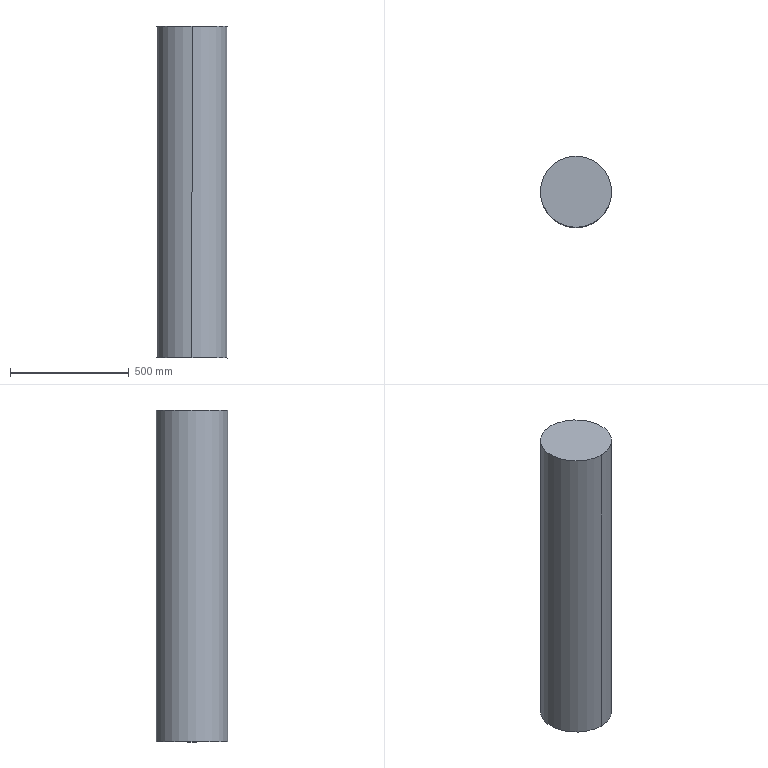Component | SolidWorks | RunningMechanism-4_Part14-1 | 1 solid | 4 faces | box 300 x 300 x 1400 mm | volume 98960169 mm3 | cylinder 2 | plane 2 | commonest cylinder face diameters 300 x2
build123d program:
from build123d import *

# Parameters (mm, degrees)
SKETCH1_R           = 150
BOSS_EXTRUDE1_DEPTH = 700


with BuildPart() as part:
    # Sketch1 → Boss-Extrude1 (new, symmetric)
    with BuildSketch(Plane(origin=(0, 0, 0), x_dir=(1, 0, 0), z_dir=(0, 1, 0))):
        with Locations(Location((0, 0, 0), (0, 0, 270))):
            Circle(SKETCH1_R)
    extrude(amount=BOSS_EXTRUDE1_DEPTH, both=True)


solid = part.part

# Placed as in the assembly
solid = solid.moved(Location((-1758.959, 55398.441, 24073.004), (90, 0, 0)))
STEP:
#1=COLOUR_RGB('',0.7922,0.8196,0.9333);
#2=FILL_AREA_STYLE_COLOUR('',#1);
#3=FILL_AREA_STYLE('',(#2));
#4=SURFACE_STYLE_FILL_AREA(#3);
#5=SURFACE_SIDE_STYLE('',(#4));
#6=SURFACE_STYLE_USAGE(.BOTH.,#5);
#7=PRESENTATION_STYLE_ASSIGNMENT((#6));
#8=CARTESIAN_POINT('',(-69.25,2175.135,920.197));
#9=VERTEX_POINT('',#8);
#10=CARTESIAN_POINT('',(-69.25,2186.947,920.197));
#11=VERTEX_POINT('',#10);
#12=CARTESIAN_POINT('',(-69.25,2181.041,920.197));
#13=DIRECTION('',(-0.0000002,-0.,-1.));
#14=DIRECTION('',(0.,-1.,0.));
#15=AXIS2_PLACEMENT_3D('',#12,#13,#14);
#16=CIRCLE('',#15,5.906);
#17=EDGE_CURVE('',#9,#11,#16,.T.);
#18=ORIENTED_EDGE('',*,*,#17,.F.);
#19=CARTESIAN_POINT('',(-69.25,2175.135,975.315));
#20=VERTEX_POINT('',#19);
#21=CARTESIAN_POINT('',(-69.25,2175.135,920.197));
#22=DIRECTION('',(0.0000002,0.,1.));
#23=VECTOR('',#22,39.37);
#24=LINE('',#21,#23);
#25=EDGE_CURVE('',#9,#20,#24,.T.);
#26=ORIENTED_EDGE('',*,*,#25,.T.);
#27=CARTESIAN_POINT('',(-69.25,2186.947,975.315));
#28=VERTEX_POINT('',#27);
#29=CARTESIAN_POINT('',(-69.25,2181.041,975.315));
#30=DIRECTION('',(-0.0000002,-0.,-1.));
#31=DIRECTION('',(0.,-1.,0.));
#32=AXIS2_PLACEMENT_3D('',#29,#30,#31);
#33=CIRCLE('',#32,5.906);
#34=EDGE_CURVE('',#20,#28,#33,.T.);
#35=ORIENTED_EDGE('',*,*,#34,.T.);
#36=CARTESIAN_POINT('',(-69.25,2186.947,920.197));
#37=DIRECTION('',(0.0000002,0.,1.));
#38=VECTOR('',#37,39.37);
#39=LINE('',#36,#38);
#40=EDGE_CURVE('',#11,#28,#39,.T.);
#41=ORIENTED_EDGE('',*,*,#40,.F.);
#42=EDGE_LOOP('',(#18,#26,#35,#41));
#43=FACE_OUTER_BOUND('',#42,.T.);
#44=CARTESIAN_POINT('',(-69.25,2181.041,920.197));
#45=DIRECTION('',(0.0000002,0.,1.));
#46=DIRECTION('',(0.,1.,0.));
#47=AXIS2_PLACEMENT_3D('',#44,#45,#46);
#48=CYLINDRICAL_SURFACE('',#47,5.906);
#49=ADVANCED_FACE('',(#43),#48,.T.);
#50=ORIENTED_EDGE('',*,*,#25,.F.);
#51=CARTESIAN_POINT('',(-69.25,2181.041,920.197));
#52=DIRECTION('',(-0.0000002,-0.,-1.));
#53=DIRECTION('',(0.,-1.,0.));
#54=AXIS2_PLACEMENT_3D('',#51,#52,#53);
#55=CIRCLE('',#54,5.906);
#56=EDGE_CURVE('',#11,#9,#55,.T.);
#57=ORIENTED_EDGE('',*,*,#56,.F.);
#58=ORIENTED_EDGE('',*,*,#40,.T.);
#59=CARTESIAN_POINT('',(-69.25,2181.041,975.315));
#60=DIRECTION('',(-0.0000002,-0.,-1.));
#61=DIRECTION('',(0.,-1.,0.));
#62=AXIS2_PLACEMENT_3D('',#59,#60,#61);
#63=CIRCLE('',#62,5.906);
#64=EDGE_CURVE('',#28,#20,#63,.T.);
#65=ORIENTED_EDGE('',*,*,#64,.T.);
#66=EDGE_LOOP('',(#50,#57,#58,#65));
#67=FACE_OUTER_BOUND('',#66,.T.);
#68=CARTESIAN_POINT('',(-69.25,2181.041,920.197));
#69=DIRECTION('',(0.0000002,0.,1.));
#70=DIRECTION('',(0.,1.,0.));
#71=AXIS2_PLACEMENT_3D('',#68,#69,#70);
#72=CYLINDRICAL_SURFACE('',#71,5.906);
#73=ADVANCED_FACE('',(#67),#72,.T.);
#74=ORIENTED_EDGE('',*,*,#56,.T.);
#75=ORIENTED_EDGE('',*,*,#17,.T.);
#76=EDGE_LOOP('',(#74,#75));
#77=FACE_OUTER_BOUND('',#76,.T.);
#78=CARTESIAN_POINT('',(-69.25,2181.041,920.197));
#79=DIRECTION('',(-0.0000002,-0.,-1.));
#80=DIRECTION('',(0.,-1.,0.));
#81=AXIS2_PLACEMENT_3D('',#78,#79,#80);
#82=PLANE('',#81);
#83=ADVANCED_FACE('',(#77),#82,.T.);
#84=ORIENTED_EDGE('',*,*,#64,.F.);
#85=ORIENTED_EDGE('',*,*,#34,.F.);
#86=EDGE_LOOP('',(#84,#85));
#87=FACE_OUTER_BOUND('',#86,.T.);
#88=CARTESIAN_POINT('',(-69.25,2181.041,975.315));
#89=DIRECTION('',(-0.0000002,-0.,-1.));
#90=DIRECTION('',(0.,-1.,0.));
#91=AXIS2_PLACEMENT_3D('',#88,#89,#90);
#92=PLANE('',#91);
#93=ADVANCED_FACE('',(#87),#92,.F.);
#94=CLOSED_SHELL('',(#49,#73,#83,#93));
#95=MANIFOLD_SOLID_BREP('',#94);
#96=STYLED_ITEM('',(#7),#95);
#97=PRESENTATION_LAYER_ASSIGNMENT('','',(#96));
#98=(LENGTH_UNIT()NAMED_UNIT(*)SI_UNIT($,.METRE.));
#99=LENGTH_MEASURE_WITH_UNIT(LENGTH_MEASURE(0.0254),#98);
#100=DIMENSIONAL_EXPONENTS(1.,0.,0.,0.,0.,0.,0.);
#101=(CONVERSION_BASED_UNIT('',#99)LENGTH_UNIT()NAMED_UNIT(#100));
#102=UNCERTAINTY_MEASURE_WITH_UNIT(LENGTH_MEASURE(0.00001),#101,'','');
#103=(NAMED_UNIT(*)PLANE_ANGLE_UNIT()SI_UNIT($,.RADIAN.));
#104=(NAMED_UNIT(*)SI_UNIT($,.STERADIAN.)SOLID_ANGLE_UNIT());
#105=(GEOMETRIC_REPRESENTATION_CONTEXT(3)GLOBAL_UNCERTAINTY_ASSIGNED_CONTEXT((#102))GLOBAL_UNIT_ASSIGNED_CONTEXT((#101,#103,#104))REPRESENTATION_CONTEXT('',''));
#106=MECHANICAL_DESIGN_GEOMETRIC_PRESENTATION_REPRESENTATION('',(#96),#105);
#107=CARTESIAN_POINT('',(0.,0.,0.));
#108=DIRECTION('',(0.,0.,1.));
#109=DIRECTION('',(1.,0.,0.));
#110=AXIS2_PLACEMENT_3D('',#107,#108,#109);
#111=(LENGTH_UNIT()NAMED_UNIT(*)SI_UNIT($,.METRE.));
#112=LENGTH_MEASURE_WITH_UNIT(LENGTH_MEASURE(0.0254),#111);
#113=DIMENSIONAL_EXPONENTS(1.,0.,0.,0.,0.,0.,0.);
#114=(CONVERSION_BASED_UNIT('',#112)LENGTH_UNIT()NAMED_UNIT(#113));
#115=UNCERTAINTY_MEASURE_WITH_UNIT(LENGTH_MEASURE(0.00001),#114,'','');
#116=(NAMED_UNIT(*)PLANE_ANGLE_UNIT()SI_UNIT($,.RADIAN.));
#117=(NAMED_UNIT(*)SI_UNIT($,.STERADIAN.)SOLID_ANGLE_UNIT());
#118=(GEOMETRIC_REPRESENTATION_CONTEXT(3)GLOBAL_UNCERTAINTY_ASSIGNED_CONTEXT((#115))GLOBAL_UNIT_ASSIGNED_CONTEXT((#114,#116,#117))REPRESENTATION_CONTEXT('',''));
#119=ADVANCED_BREP_SHAPE_REPRESENTATION('',(#95,#110),#118);